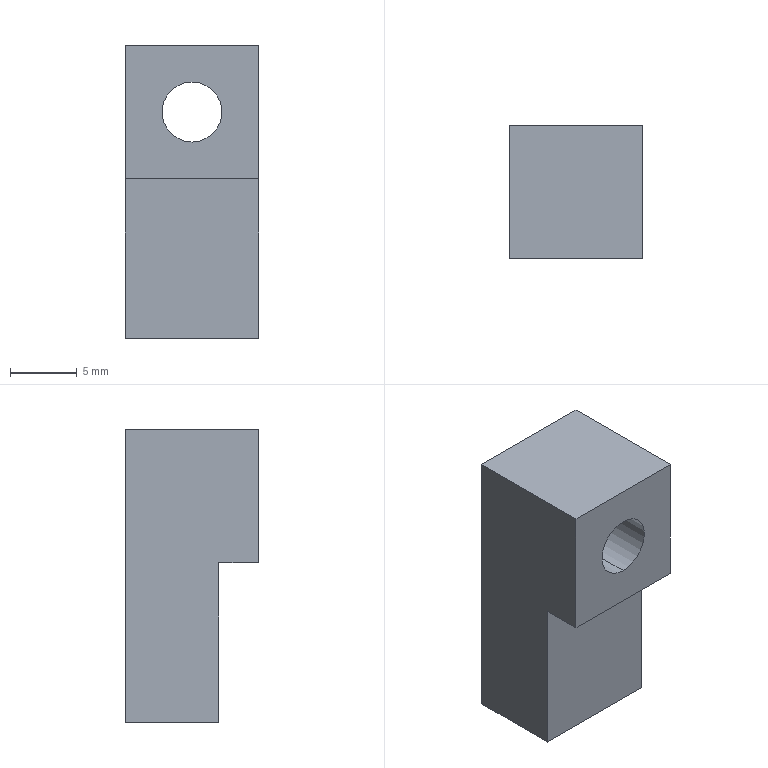Component | SolidWorks | 09HHHHHH7-1 | 1 solid | 13 faces | box 10 x 10 x 22 mm | volume 1523 mm3 | plane 9 | cylinder 4 | commonest cylinder face diameters 8 x2 4.5 x2
build123d program:
from build123d import *

# Parameters (mm, degrees)
SKETCH1_W                                            = 10
SKETCH1_H                                            = 10
BOSS_EXTRUDE1_DEPTH                                  = 30
SKETCH2_W                                            = 20
SKETCH2_H                                            = 3
CUT_EXTRUDE1_DEPTH                                   = 284.768
HOLE_SIZE_ACCORDING_TO_THE_TYPE_OF_HEXAG_D           = 4.5
HOLE_SIZE_ACCORDING_TO_THE_TYPE_OF_HEXAG_CBORE_D     = 8
HOLE_SIZE_ACCORDING_TO_THE_TYPE_OF_HEXAG_CBORE_DEPTH = 4.6
MOVE_FACE1_BY                                        = 8


with BuildPart() as part:
    # Sketch1 → Boss-Extrude1 (new body)
    with BuildSketch(Plane.XY):
        with Locations((-587.359, -277)):
            Rectangle(SKETCH1_W, SKETCH1_H)
    extrude(amount=-BOSS_EXTRUDE1_DEPTH)

    # Sketch2 → Cut-Extrude1 (cut, through all)
    with BuildSketch(Plane(origin=(-582.359, 0, 0), x_dir=(0, 0, -1), z_dir=(1, 0, 0))):
        with Locations((20, -280.5)):
            Rectangle(SKETCH2_W, SKETCH2_H)
    extrude(amount=-CUT_EXTRUDE1_DEPTH, mode=Mode.SUBTRACT)

    # Hole Size according to the type of hexag (through all)
    with Locations(Plane(origin=(0, -272, 0), x_dir=(1, 0, 0), z_dir=(0, 1, 0))):
        with Locations((-587.359, 5)):
            CounterBoreHole(HOLE_SIZE_ACCORDING_TO_THE_TYPE_OF_HEXAG_D / 2, HOLE_SIZE_ACCORDING_TO_THE_TYPE_OF_HEXAG_CBORE_D / 2, HOLE_SIZE_ACCORDING_TO_THE_TYPE_OF_HEXAG_CBORE_DEPTH)

    # Move Face1: a face moved inward by 8.0
    extrude(part.faces().sort_by_distance((-587.359, -275.5, -30))[0], amount=MOVE_FACE1_BY, dir=(0, 0, 1), mode=Mode.SUBTRACT)


solid = part.part

# Placed as in the assembly
solid = solid.moved(Location((-10.581, 13.617, 8.844), (0, 0, 0)))
STEP:
#1=COLOUR_RGB('',0.7922,0.8196,0.9333);
#2=FILL_AREA_STYLE_COLOUR('',#1);
#3=FILL_AREA_STYLE('',(#2));
#4=SURFACE_STYLE_FILL_AREA(#3);
#5=SURFACE_SIDE_STYLE('',(#4));
#6=SURFACE_STYLE_USAGE(.BOTH.,#5);
#7=PRESENTATION_STYLE_ASSIGNMENT((#6));
#8=CARTESIAN_POINT('',(-23.541,-10.354,-0.006151));
#9=VERTEX_POINT('',#8);
#10=CARTESIAN_POINT('',(-23.541,-10.354,0.3088));
#11=VERTEX_POINT('',#10);
#12=CARTESIAN_POINT('',(-23.541,-10.354,0.1513));
#13=DIRECTION('',(0.,1.,0.));
#14=DIRECTION('',(0.,0.,1.));
#15=AXIS2_PLACEMENT_3D('',#12,#13,#14);
#16=CIRCLE('',#15,0.1575);
#17=EDGE_CURVE('',#9,#11,#16,.T.);
#18=ORIENTED_EDGE('',*,*,#17,.F.);
#19=CARTESIAN_POINT('',(-23.541,-10.173,-0.006151));
#20=VERTEX_POINT('',#19);
#21=CARTESIAN_POINT('',(-23.541,-10.173,-0.006151));
#22=DIRECTION('',(0.,1.,0.));
#23=VECTOR('',#22,39.37);
#24=LINE('',#21,#23);
#25=EDGE_CURVE('',#9,#20,#24,.T.);
#26=ORIENTED_EDGE('',*,*,#25,.T.);
#27=CARTESIAN_POINT('',(-23.541,-10.173,0.3088));
#28=VERTEX_POINT('',#27);
#29=CARTESIAN_POINT('',(-23.541,-10.173,0.1513));
#30=DIRECTION('',(0.,1.,0.));
#31=DIRECTION('',(0.,0.,1.));
#32=AXIS2_PLACEMENT_3D('',#29,#30,#31);
#33=CIRCLE('',#32,0.1575);
#34=EDGE_CURVE('',#20,#28,#33,.T.);
#35=ORIENTED_EDGE('',*,*,#34,.T.);
#36=CARTESIAN_POINT('',(-23.541,-10.173,0.3088));
#37=DIRECTION('',(0.,1.,0.));
#38=VECTOR('',#37,39.37);
#39=LINE('',#36,#38);
#40=EDGE_CURVE('',#11,#28,#39,.T.);
#41=ORIENTED_EDGE('',*,*,#40,.F.);
#42=EDGE_LOOP('',(#18,#26,#35,#41));
#43=FACE_OUTER_BOUND('',#42,.T.);
#44=CARTESIAN_POINT('',(-23.541,-10.173,0.1513));
#45=DIRECTION('',(0.,1.,0.));
#46=DIRECTION('',(0.,0.,1.));
#47=AXIS2_PLACEMENT_3D('',#44,#45,#46);
#48=CYLINDRICAL_SURFACE('',#47,0.1575);
#49=ADVANCED_FACE('',(#43),#48,.F.);
#50=CARTESIAN_POINT('',(-23.541,-10.566,0.06275));
#51=VERTEX_POINT('',#50);
#52=CARTESIAN_POINT('',(-23.541,-10.566,0.2399));
#53=VERTEX_POINT('',#52);
#54=CARTESIAN_POINT('',(-23.541,-10.566,0.1513));
#55=DIRECTION('',(0.,1.,0.));
#56=DIRECTION('',(0.,0.,1.));
#57=AXIS2_PLACEMENT_3D('',#54,#55,#56);
#58=CIRCLE('',#57,0.08858);
#59=EDGE_CURVE('',#51,#53,#58,.T.);
#60=ORIENTED_EDGE('',*,*,#59,.F.);
#61=CARTESIAN_POINT('',(-23.541,-10.354,0.06275));
#62=VERTEX_POINT('',#61);
#63=CARTESIAN_POINT('',(-23.541,-10.173,0.06275));
#64=DIRECTION('',(0.,1.,0.));
#65=VECTOR('',#64,39.37);
#66=LINE('',#63,#65);
#67=EDGE_CURVE('',#51,#62,#66,.T.);
#68=ORIENTED_EDGE('',*,*,#67,.T.);
#69=CARTESIAN_POINT('',(-23.541,-10.354,0.2399));
#70=VERTEX_POINT('',#69);
#71=CARTESIAN_POINT('',(-23.541,-10.354,0.1513));
#72=DIRECTION('',(0.,1.,0.));
#73=DIRECTION('',(0.,0.,1.));
#74=AXIS2_PLACEMENT_3D('',#71,#72,#73);
#75=CIRCLE('',#74,0.08858);
#76=EDGE_CURVE('',#62,#70,#75,.T.);
#77=ORIENTED_EDGE('',*,*,#76,.T.);
#78=CARTESIAN_POINT('',(-23.541,-10.173,0.2399));
#79=DIRECTION('',(0.,1.,0.));
#80=VECTOR('',#79,39.37);
#81=LINE('',#78,#80);
#82=EDGE_CURVE('',#53,#70,#81,.T.);
#83=ORIENTED_EDGE('',*,*,#82,.F.);
#84=EDGE_LOOP('',(#60,#68,#77,#83));
#85=FACE_OUTER_BOUND('',#84,.T.);
#86=CARTESIAN_POINT('',(-23.541,-10.173,0.1513));
#87=DIRECTION('',(0.,1.,0.));
#88=DIRECTION('',(0.,0.,1.));
#89=AXIS2_PLACEMENT_3D('',#86,#87,#88);
#90=CYLINDRICAL_SURFACE('',#89,0.08858);
#91=ADVANCED_FACE('',(#85),#90,.F.);
#92=CARTESIAN_POINT('',(-23.344,-10.448,-0.04552));
#93=VERTEX_POINT('',#92);
#94=CARTESIAN_POINT('',(-23.344,-10.566,-0.04552));
#95=VERTEX_POINT('',#94);
#96=CARTESIAN_POINT('',(-23.344,-10.566,-0.04552));
#97=DIRECTION('',(0.,-1.,0.));
#98=VECTOR('',#97,39.37);
#99=LINE('',#96,#98);
#100=EDGE_CURVE('',#93,#95,#99,.T.);
#101=ORIENTED_EDGE('',*,*,#100,.F.);
#102=CARTESIAN_POINT('',(-23.344,-10.448,-0.518));
#103=VERTEX_POINT('',#102);
#104=CARTESIAN_POINT('',(-23.344,-10.448,-0.8329));
#105=DIRECTION('',(0.,0.,1.));
#106=VECTOR('',#105,39.37);
#107=LINE('',#104,#106);
#108=EDGE_CURVE('',#103,#93,#107,.T.);
#109=ORIENTED_EDGE('',*,*,#108,.F.);
#110=CARTESIAN_POINT('',(-23.344,-10.173,-0.518));
#111=VERTEX_POINT('',#110);
#112=CARTESIAN_POINT('',(-23.344,0.5361,-0.518));
#113=DIRECTION('',(0.,1.,0.));
#114=VECTOR('',#113,39.37);
#115=LINE('',#112,#114);
#116=EDGE_CURVE('',#103,#111,#115,.T.);
#117=ORIENTED_EDGE('',*,*,#116,.T.);
#118=CARTESIAN_POINT('',(-23.344,-10.173,0.3482));
#119=VERTEX_POINT('',#118);
#120=CARTESIAN_POINT('',(-23.344,-10.173,-0.8329));
#121=DIRECTION('',(0.,0.,1.));
#122=VECTOR('',#121,39.37);
#123=LINE('',#120,#122);
#124=EDGE_CURVE('',#111,#119,#123,.T.);
#125=ORIENTED_EDGE('',*,*,#124,.T.);
#126=CARTESIAN_POINT('',(-23.344,-10.566,0.3482));
#127=VERTEX_POINT('',#126);
#128=CARTESIAN_POINT('',(-23.344,-10.566,0.3482));
#129=DIRECTION('',(0.,1.,0.));
#130=VECTOR('',#129,39.37);
#131=LINE('',#128,#130);
#132=EDGE_CURVE('',#127,#119,#131,.T.);
#133=ORIENTED_EDGE('',*,*,#132,.F.);
#134=CARTESIAN_POINT('',(-23.344,-10.566,-0.8329));
#135=DIRECTION('',(0.,0.,1.));
#136=VECTOR('',#135,39.37);
#137=LINE('',#134,#136);
#138=EDGE_CURVE('',#95,#127,#137,.T.);
#139=ORIENTED_EDGE('',*,*,#138,.F.);
#140=EDGE_LOOP('',(#101,#109,#117,#125,#133,#139));
#141=FACE_OUTER_BOUND('',#140,.T.);
#142=CARTESIAN_POINT('',(-23.344,-10.566,-0.8329));
#143=DIRECTION('',(1.,0.,0.));
#144=DIRECTION('',(0.,0.,-1.));
#145=AXIS2_PLACEMENT_3D('',#142,#143,#144);
#146=PLANE('',#145);
#147=ADVANCED_FACE('',(#141),#146,.T.);
#148=CARTESIAN_POINT('',(-23.541,-10.566,0.1513));
#149=DIRECTION('',(0.,1.,0.));
#150=DIRECTION('',(0.,0.,1.));
#151=AXIS2_PLACEMENT_3D('',#148,#149,#150);
#152=CIRCLE('',#151,0.08858);
#153=EDGE_CURVE('',#53,#51,#152,.T.);
#154=ORIENTED_EDGE('',*,*,#153,.T.);
#155=ORIENTED_EDGE('',*,*,#59,.T.);
#156=EDGE_LOOP('',(#154,#155));
#157=FACE_BOUND('',#156,.T.);
#158=CARTESIAN_POINT('',(-23.738,-10.566,-0.04552));
#159=VERTEX_POINT('',#158);
#160=CARTESIAN_POINT('',(-23.738,-10.566,-0.04552));
#161=DIRECTION('',(1.,0.,0.));
#162=VECTOR('',#161,39.37);
#163=LINE('',#160,#162);
#164=EDGE_CURVE('',#159,#95,#163,.T.);
#165=ORIENTED_EDGE('',*,*,#164,.T.);
#166=ORIENTED_EDGE('',*,*,#138,.T.);
#167=CARTESIAN_POINT('',(-23.738,-10.566,0.3482));
#168=VERTEX_POINT('',#167);
#169=CARTESIAN_POINT('',(-23.344,-10.566,0.3482));
#170=DIRECTION('',(1.,0.,0.));
#171=VECTOR('',#170,39.37);
#172=LINE('',#169,#171);
#173=EDGE_CURVE('',#168,#127,#172,.T.);
#174=ORIENTED_EDGE('',*,*,#173,.F.);
#175=CARTESIAN_POINT('',(-23.738,-10.566,-0.8329));
#176=DIRECTION('',(0.,0.,1.));
#177=VECTOR('',#176,39.37);
#178=LINE('',#175,#177);
#179=EDGE_CURVE('',#159,#168,#178,.T.);
#180=ORIENTED_EDGE('',*,*,#179,.F.);
#181=EDGE_LOOP('',(#165,#166,#174,#180));
#182=FACE_OUTER_BOUND('',#181,.T.);
#183=CARTESIAN_POINT('',(-23.344,-10.566,-0.8329));
#184=DIRECTION('',(0.,-1.,0.));
#185=DIRECTION('',(0.,0.,-1.));
#186=AXIS2_PLACEMENT_3D('',#183,#184,#185);
#187=PLANE('',#186);
#188=ADVANCED_FACE('',(#157,#182),#187,.T.);
#189=CARTESIAN_POINT('',(-23.738,-10.448,-0.04552));
#190=VERTEX_POINT('',#189);
#191=CARTESIAN_POINT('',(-23.738,-10.566,-0.04552));
#192=DIRECTION('',(0.,-1.,0.));
#193=VECTOR('',#192,39.37);
#194=LINE('',#191,#193);
#195=EDGE_CURVE('',#190,#159,#194,.T.);
#196=ORIENTED_EDGE('',*,*,#195,.T.);
#197=ORIENTED_EDGE('',*,*,#179,.T.);
#198=CARTESIAN_POINT('',(-23.738,-10.173,0.3482));
#199=VERTEX_POINT('',#198);
#200=CARTESIAN_POINT('',(-23.738,-10.566,0.3482));
#201=DIRECTION('',(0.,-1.,0.));
#202=VECTOR('',#201,39.37);
#203=LINE('',#200,#202);
#204=EDGE_CURVE('',#199,#168,#203,.T.);
#205=ORIENTED_EDGE('',*,*,#204,.F.);
#206=CARTESIAN_POINT('',(-23.738,-10.173,-0.518));
#207=VERTEX_POINT('',#206);
#208=CARTESIAN_POINT('',(-23.738,-10.173,-0.8329));
#209=DIRECTION('',(0.,0.,1.));
#210=VECTOR('',#209,39.37);
#211=LINE('',#208,#210);
#212=EDGE_CURVE('',#207,#199,#211,.T.);
#213=ORIENTED_EDGE('',*,*,#212,.F.);
#214=CARTESIAN_POINT('',(-23.738,-10.448,-0.518));
#215=VERTEX_POINT('',#214);
#216=CARTESIAN_POINT('',(-23.738,0.5361,-0.518));
#217=DIRECTION('',(0.,-1.,0.));
#218=VECTOR('',#217,39.37);
#219=LINE('',#216,#218);
#220=EDGE_CURVE('',#207,#215,#219,.T.);
#221=ORIENTED_EDGE('',*,*,#220,.T.);
#222=CARTESIAN_POINT('',(-23.738,-10.448,-0.8329));
#223=DIRECTION('',(0.,0.,1.));
#224=VECTOR('',#223,39.37);
#225=LINE('',#222,#224);
#226=EDGE_CURVE('',#215,#190,#225,.T.);
#227=ORIENTED_EDGE('',*,*,#226,.T.);
#228=EDGE_LOOP('',(#196,#197,#205,#213,#221,#227));
#229=FACE_OUTER_BOUND('',#228,.T.);
#230=CARTESIAN_POINT('',(-23.738,-10.566,-0.8329));
#231=DIRECTION('',(-1.,0.,0.));
#232=DIRECTION('',(0.,0.,1.));
#233=AXIS2_PLACEMENT_3D('',#230,#231,#232);
#234=PLANE('',#233);
#235=ADVANCED_FACE('',(#229),#234,.T.);
#236=CARTESIAN_POINT('',(-23.541,-10.173,0.1513));
#237=DIRECTION('',(0.,1.,0.));
#238=DIRECTION('',(0.,0.,1.));
#239=AXIS2_PLACEMENT_3D('',#236,#237,#238);
#240=CIRCLE('',#239,0.1575);
#241=EDGE_CURVE('',#28,#20,#240,.T.);
#242=ORIENTED_EDGE('',*,*,#241,.F.);
#243=ORIENTED_EDGE('',*,*,#34,.F.);
#244=EDGE_LOOP('',(#242,#243));
#245=FACE_BOUND('',#244,.T.);
#246=CARTESIAN_POINT('',(-23.344,-10.173,0.3482));
#247=DIRECTION('',(-1.,0.,0.));
#248=VECTOR('',#247,39.37);
#249=LINE('',#246,#248);
#250=EDGE_CURVE('',#119,#199,#249,.T.);
#251=ORIENTED_EDGE('',*,*,#250,.F.);
#252=ORIENTED_EDGE('',*,*,#124,.F.);
#253=CARTESIAN_POINT('',(-0.4166,-10.173,-0.518));
#254=DIRECTION('',(-1.,0.,0.));
#255=VECTOR('',#254,39.37);
#256=LINE('',#253,#255);
#257=EDGE_CURVE('',#111,#207,#256,.T.);
#258=ORIENTED_EDGE('',*,*,#257,.T.);
#259=ORIENTED_EDGE('',*,*,#212,.T.);
#260=EDGE_LOOP('',(#251,#252,#258,#259));
#261=FACE_OUTER_BOUND('',#260,.T.);
#262=CARTESIAN_POINT('',(-23.344,-10.173,-0.8329));
#263=DIRECTION('',(0.,1.,0.));
#264=DIRECTION('',(0.,0.,1.));
#265=AXIS2_PLACEMENT_3D('',#262,#263,#264);
#266=PLANE('',#265);
#267=ADVANCED_FACE('',(#245,#261),#266,.T.);
#268=ORIENTED_EDGE('',*,*,#116,.F.);
#269=CARTESIAN_POINT('',(-23.738,-10.448,-0.518));
#270=DIRECTION('',(1.,0.,0.));
#271=VECTOR('',#270,39.37);
#272=LINE('',#269,#271);
#273=EDGE_CURVE('',#215,#103,#272,.T.);
#274=ORIENTED_EDGE('',*,*,#273,.F.);
#275=ORIENTED_EDGE('',*,*,#220,.F.);
#276=ORIENTED_EDGE('',*,*,#257,.F.);
#277=EDGE_LOOP('',(#268,#274,#275,#276));
#278=FACE_OUTER_BOUND('',#277,.T.);
#279=CARTESIAN_POINT('',(-0.4166,0.5361,-0.518));
#280=DIRECTION('',(0.,0.,1.));
#281=DIRECTION('',(1.,0.,0.));
#282=AXIS2_PLACEMENT_3D('',#279,#280,#281);
#283=PLANE('',#282);
#284=ADVANCED_FACE('',(#278),#283,.F.);
#285=ORIENTED_EDGE('',*,*,#132,.T.);
#286=ORIENTED_EDGE('',*,*,#250,.T.);
#287=ORIENTED_EDGE('',*,*,#204,.T.);
#288=ORIENTED_EDGE('',*,*,#173,.T.);
#289=EDGE_LOOP('',(#285,#286,#287,#288));
#290=FACE_OUTER_BOUND('',#289,.T.);
#291=CARTESIAN_POINT('',(-0.4166,0.5361,0.3482));
#292=DIRECTION('',(0.,0.,1.));
#293=DIRECTION('',(1.,0.,0.));
#294=AXIS2_PLACEMENT_3D('',#291,#292,#293);
#295=PLANE('',#294);
#296=ADVANCED_FACE('',(#290),#295,.T.);
#297=ORIENTED_EDGE('',*,*,#100,.T.);
#298=ORIENTED_EDGE('',*,*,#164,.F.);
#299=ORIENTED_EDGE('',*,*,#195,.F.);
#300=CARTESIAN_POINT('',(-23.738,-10.448,-0.04552));
#301=DIRECTION('',(1.,0.,0.));
#302=VECTOR('',#301,39.37);
#303=LINE('',#300,#302);
#304=EDGE_CURVE('',#190,#93,#303,.T.);
#305=ORIENTED_EDGE('',*,*,#304,.T.);
#306=EDGE_LOOP('',(#297,#298,#299,#305));
#307=FACE_OUTER_BOUND('',#306,.T.);
#308=CARTESIAN_POINT('',(-23.738,-10.566,-0.04552));
#309=DIRECTION('',(0.,0.,1.));
#310=DIRECTION('',(1.,0.,0.));
#311=AXIS2_PLACEMENT_3D('',#308,#309,#310);
#312=PLANE('',#311);
#313=ADVANCED_FACE('',(#307),#312,.F.);
#314=ORIENTED_EDGE('',*,*,#108,.T.);
#315=ORIENTED_EDGE('',*,*,#304,.F.);
#316=ORIENTED_EDGE('',*,*,#226,.F.);
#317=ORIENTED_EDGE('',*,*,#273,.T.);
#318=EDGE_LOOP('',(#314,#315,#316,#317));
#319=FACE_OUTER_BOUND('',#318,.T.);
#320=CARTESIAN_POINT('',(-23.738,-10.448,-0.8329));
#321=DIRECTION('',(0.,1.,0.));
#322=DIRECTION('',(0.,0.,1.));
#323=AXIS2_PLACEMENT_3D('',#320,#321,#322);
#324=PLANE('',#323);
#325=ADVANCED_FACE('',(#319),#324,.F.);
#326=ORIENTED_EDGE('',*,*,#67,.F.);
#327=ORIENTED_EDGE('',*,*,#153,.F.);
#328=ORIENTED_EDGE('',*,*,#82,.T.);
#329=CARTESIAN_POINT('',(-23.541,-10.354,0.1513));
#330=DIRECTION('',(0.,1.,0.));
#331=DIRECTION('',(0.,0.,1.));
#332=AXIS2_PLACEMENT_3D('',#329,#330,#331);
#333=CIRCLE('',#332,0.08858);
#334=EDGE_CURVE('',#70,#62,#333,.T.);
#335=ORIENTED_EDGE('',*,*,#334,.T.);
#336=EDGE_LOOP('',(#326,#327,#328,#335));
#337=FACE_OUTER_BOUND('',#336,.T.);
#338=CARTESIAN_POINT('',(-23.541,-10.173,0.1513));
#339=DIRECTION('',(0.,1.,0.));
#340=DIRECTION('',(0.,0.,1.));
#341=AXIS2_PLACEMENT_3D('',#338,#339,#340);
#342=CYLINDRICAL_SURFACE('',#341,0.08858);
#343=ADVANCED_FACE('',(#337),#342,.F.);
#344=ORIENTED_EDGE('',*,*,#334,.F.);
#345=ORIENTED_EDGE('',*,*,#76,.F.);
#346=EDGE_LOOP('',(#344,#345));
#347=FACE_BOUND('',#346,.T.);
#348=CARTESIAN_POINT('',(-23.541,-10.354,0.1513));
#349=DIRECTION('',(0.,1.,0.));
#350=DIRECTION('',(0.,0.,1.));
#351=AXIS2_PLACEMENT_3D('',#348,#349,#350);
#352=CIRCLE('',#351,0.1575);
#353=EDGE_CURVE('',#11,#9,#352,.T.);
#354=ORIENTED_EDGE('',*,*,#353,.T.);
#355=ORIENTED_EDGE('',*,*,#17,.T.);
#356=EDGE_LOOP('',(#354,#355));
#357=FACE_OUTER_BOUND('',#356,.T.);
#358=CARTESIAN_POINT('',(-23.452,-10.354,0.1513));
#359=DIRECTION('',(0.,-1.,0.));
#360=DIRECTION('',(0.,0.,-1.));
#361=AXIS2_PLACEMENT_3D('',#358,#359,#360);
#362=PLANE('',#361);
#363=ADVANCED_FACE('',(#347,#357),#362,.F.);
#364=ORIENTED_EDGE('',*,*,#25,.F.);
#365=ORIENTED_EDGE('',*,*,#353,.F.);
#366=ORIENTED_EDGE('',*,*,#40,.T.);
#367=ORIENTED_EDGE('',*,*,#241,.T.);
#368=EDGE_LOOP('',(#364,#365,#366,#367));
#369=FACE_OUTER_BOUND('',#368,.T.);
#370=CARTESIAN_POINT('',(-23.541,-10.173,0.1513));
#371=DIRECTION('',(0.,1.,0.));
#372=DIRECTION('',(0.,0.,1.));
#373=AXIS2_PLACEMENT_3D('',#370,#371,#372);
#374=CYLINDRICAL_SURFACE('',#373,0.1575);
#375=ADVANCED_FACE('',(#369),#374,.F.);
#376=CLOSED_SHELL('',(#49,#91,#147,#188,#235,#267,#284,#296,#313,#325,#343,#363,#375));
#377=MANIFOLD_SOLID_BREP('',#376);
#378=STYLED_ITEM('',(#7),#377);
#379=PRESENTATION_LAYER_ASSIGNMENT('','',(#378));
#380=CARTESIAN_POINT('',(0.,0.,0.));
#381=DIRECTION('',(0.,0.,1.));
#382=DIRECTION('',(1.,0.,0.));
#383=AXIS2_PLACEMENT_3D('',#380,#381,#382);
#384=(LENGTH_UNIT()NAMED_UNIT(*)SI_UNIT($,.METRE.));
#385=LENGTH_MEASURE_WITH_UNIT(LENGTH_MEASURE(0.0254),#384);
#386=DIMENSIONAL_EXPONENTS(1.,0.,0.,0.,0.,0.,0.);
#387=(CONVERSION_BASED_UNIT('',#385)LENGTH_UNIT()NAMED_UNIT(#386));
#388=UNCERTAINTY_MEASURE_WITH_UNIT(LENGTH_MEASURE(0.00001),#387,'','');
#389=(NAMED_UNIT(*)PLANE_ANGLE_UNIT()SI_UNIT($,.RADIAN.));
#390=(NAMED_UNIT(*)SI_UNIT($,.STERADIAN.)SOLID_ANGLE_UNIT());
#391=(GEOMETRIC_REPRESENTATION_CONTEXT(3)GLOBAL_UNCERTAINTY_ASSIGNED_CONTEXT((#388))GLOBAL_UNIT_ASSIGNED_CONTEXT((#387,#389,#390))REPRESENTATION_CONTEXT('',''));
#392=ADVANCED_BREP_SHAPE_REPRESENTATION('',(#377,#383),#391);
#393=(LENGTH_UNIT()NAMED_UNIT(*)SI_UNIT($,.METRE.));
#394=LENGTH_MEASURE_WITH_UNIT(LENGTH_MEASURE(0.0254),#393);
#395=DIMENSIONAL_EXPONENTS(1.,0.,0.,0.,0.,0.,0.);
#396=(CONVERSION_BASED_UNIT('',#394)LENGTH_UNIT()NAMED_UNIT(#395));
#397=UNCERTAINTY_MEASURE_WITH_UNIT(LENGTH_MEASURE(0.00001),#396,'','');
#398=(NAMED_UNIT(*)PLANE_ANGLE_UNIT()SI_UNIT($,.RADIAN.));
#399=(NAMED_UNIT(*)SI_UNIT($,.STERADIAN.)SOLID_ANGLE_UNIT());
#400=(GEOMETRIC_REPRESENTATION_CONTEXT(3)GLOBAL_UNCERTAINTY_ASSIGNED_CONTEXT((#397))GLOBAL_UNIT_ASSIGNED_CONTEXT((#396,#398,#399))REPRESENTATION_CONTEXT('',''));
#401=MECHANICAL_DESIGN_GEOMETRIC_PRESENTATION_REPRESENTATION('',(#378),#400);